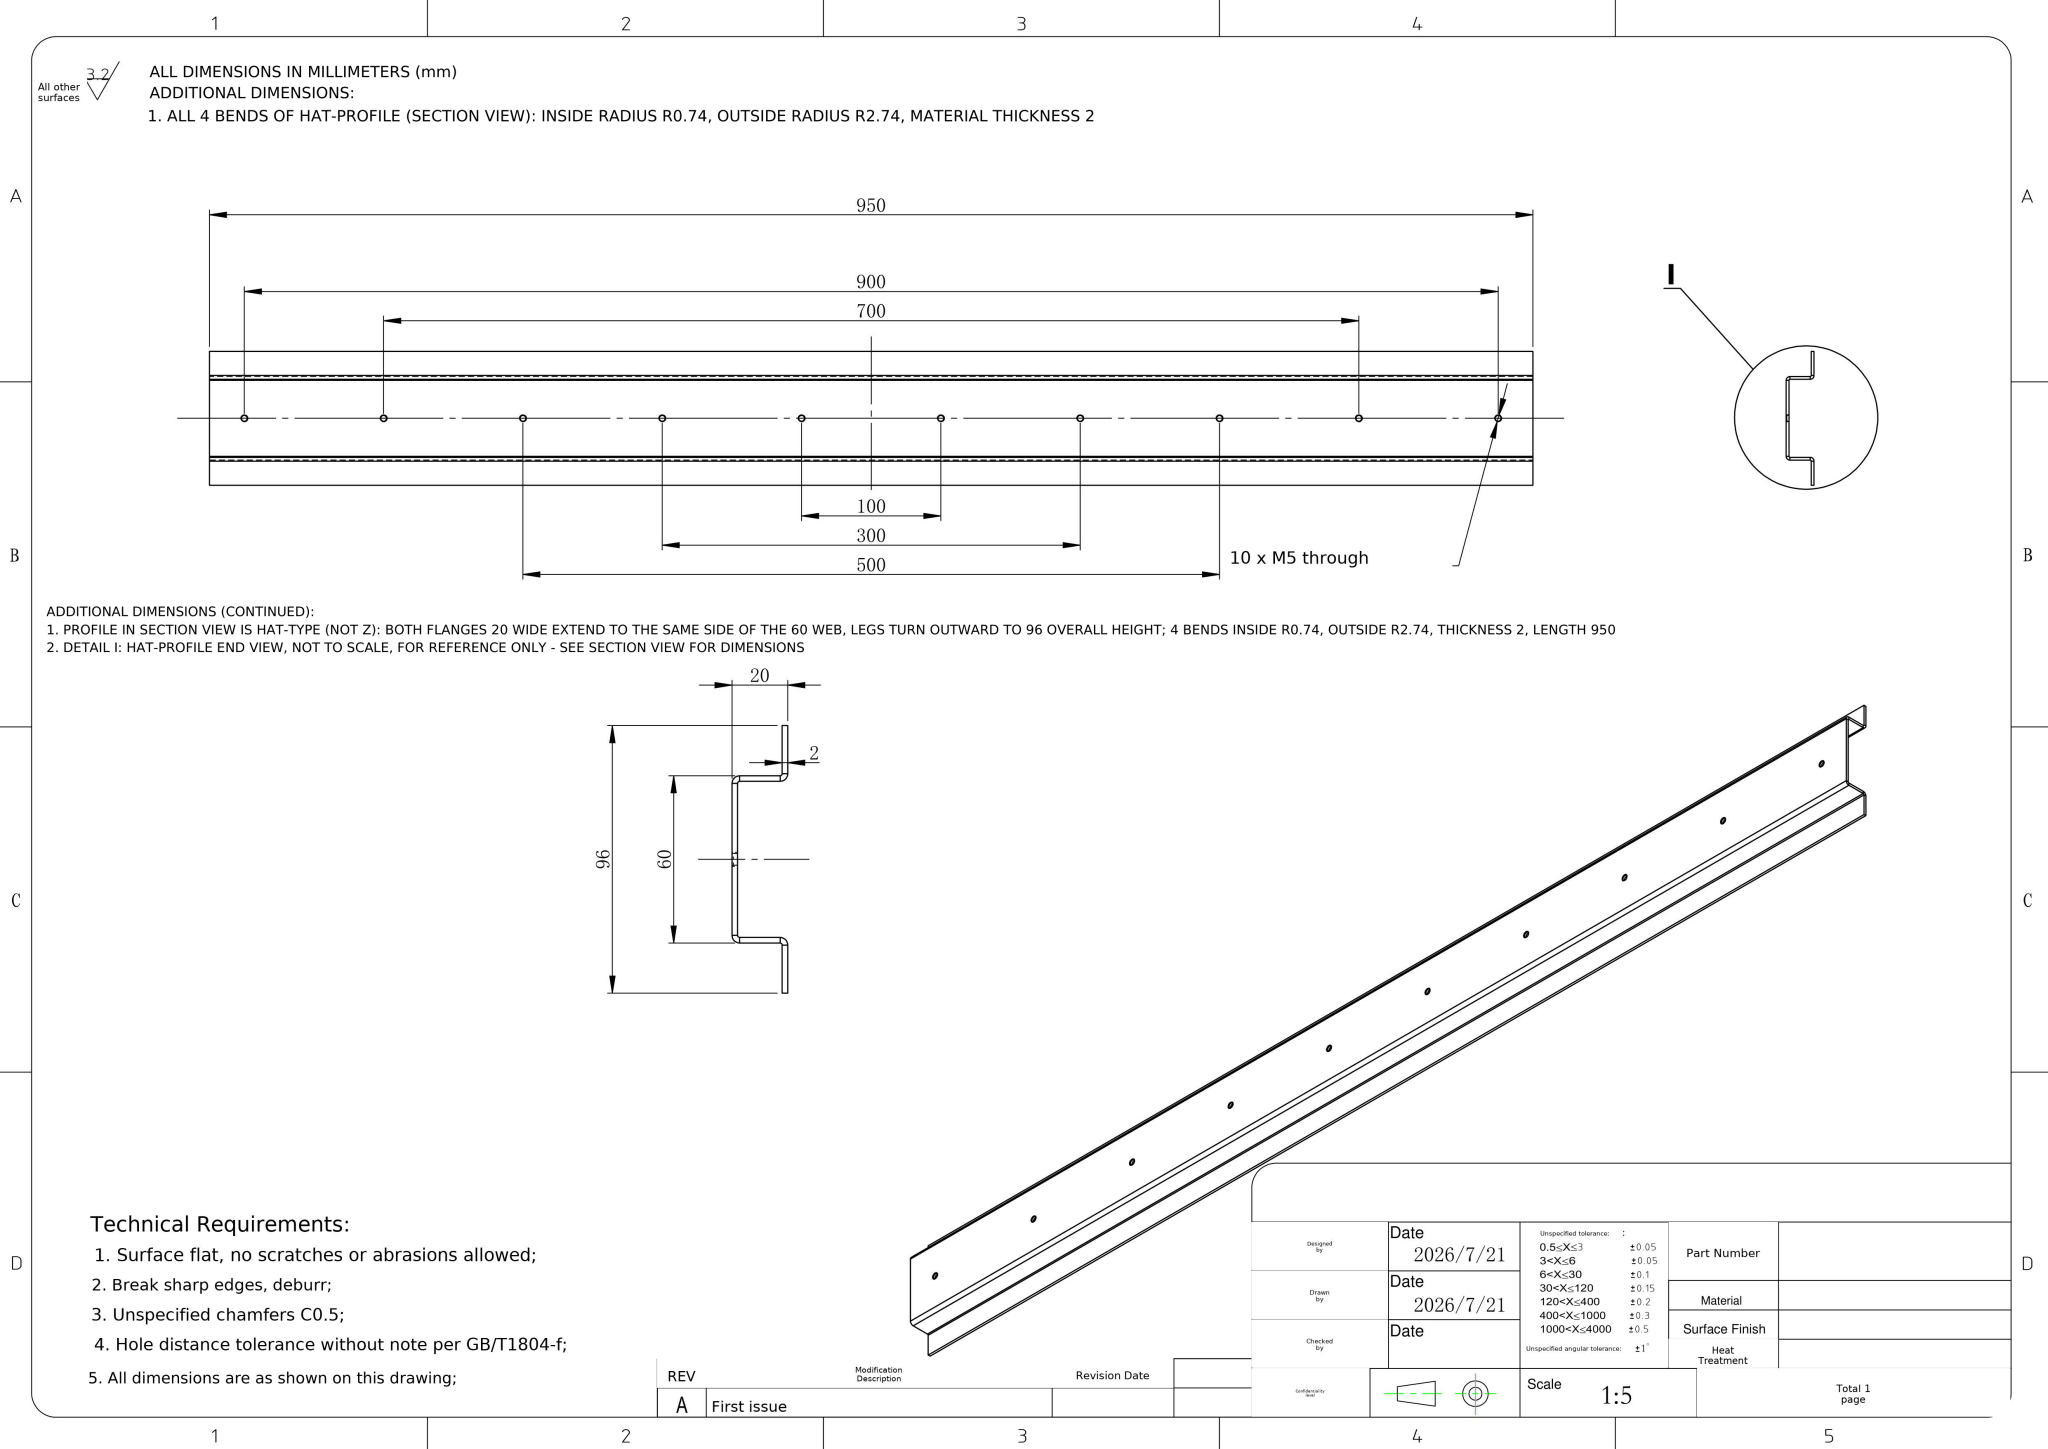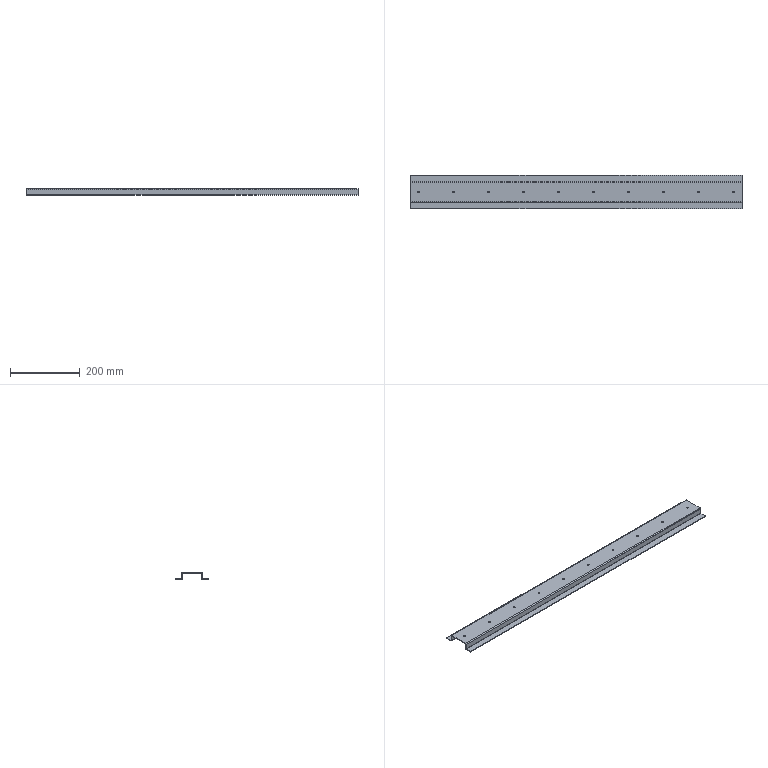Part | NX | mm | 1 solid | 78 faces | box 950 x 96 x 20 mm | volume 244845 mm3 | plane 30 | cylinder 28 | cone 20 | commonest cylinder face diameters 4.2 x20 5.473 x4 1.473 x4